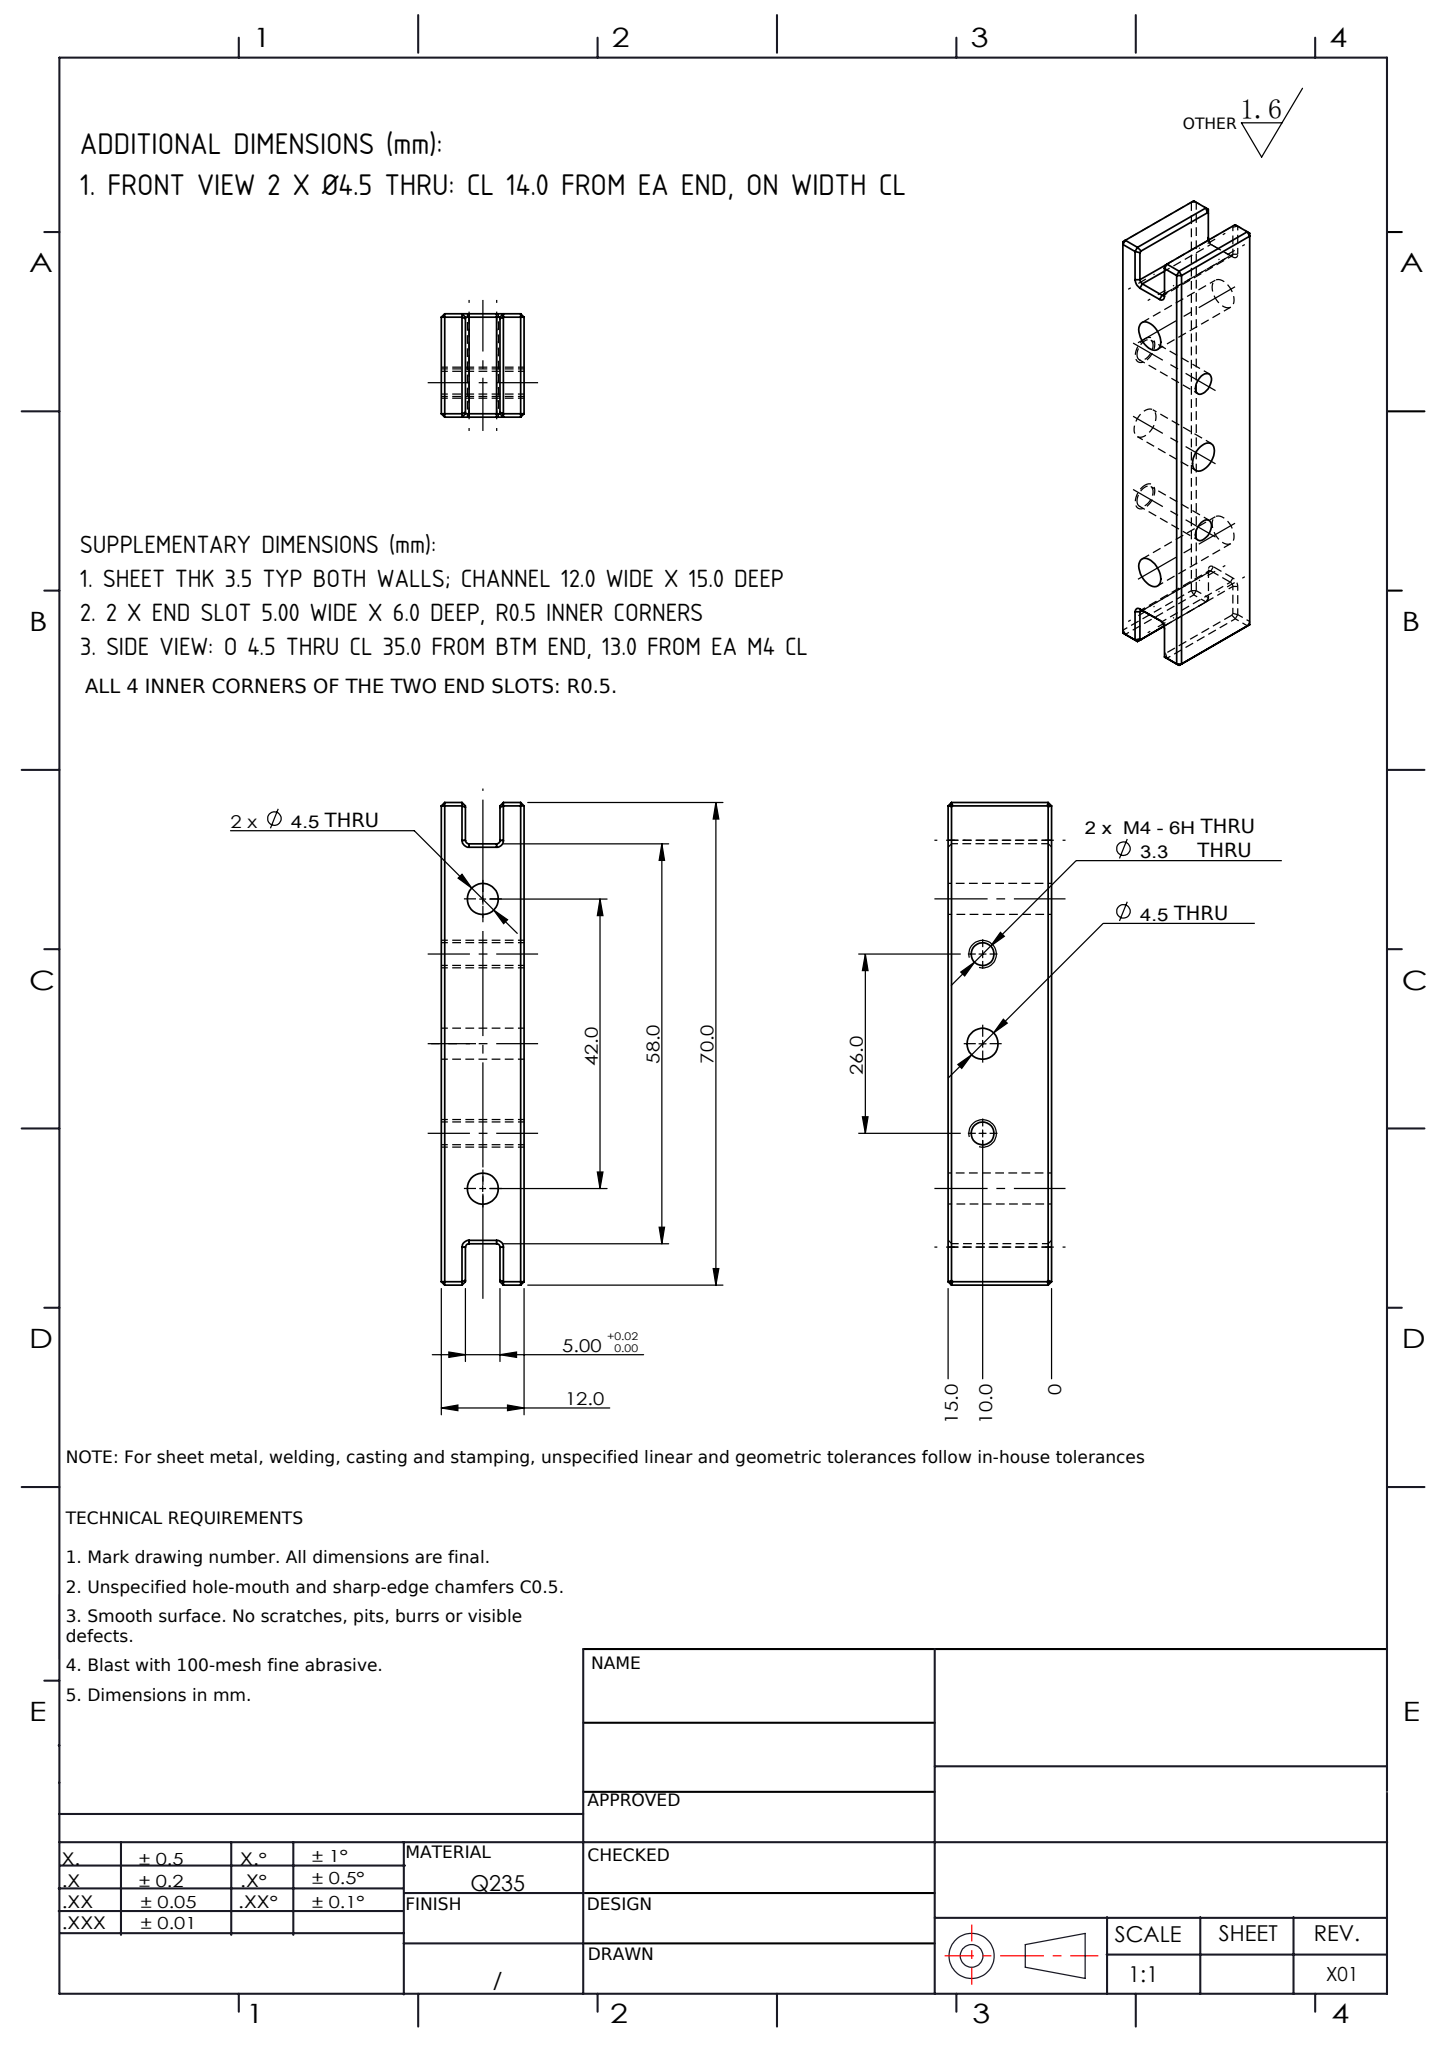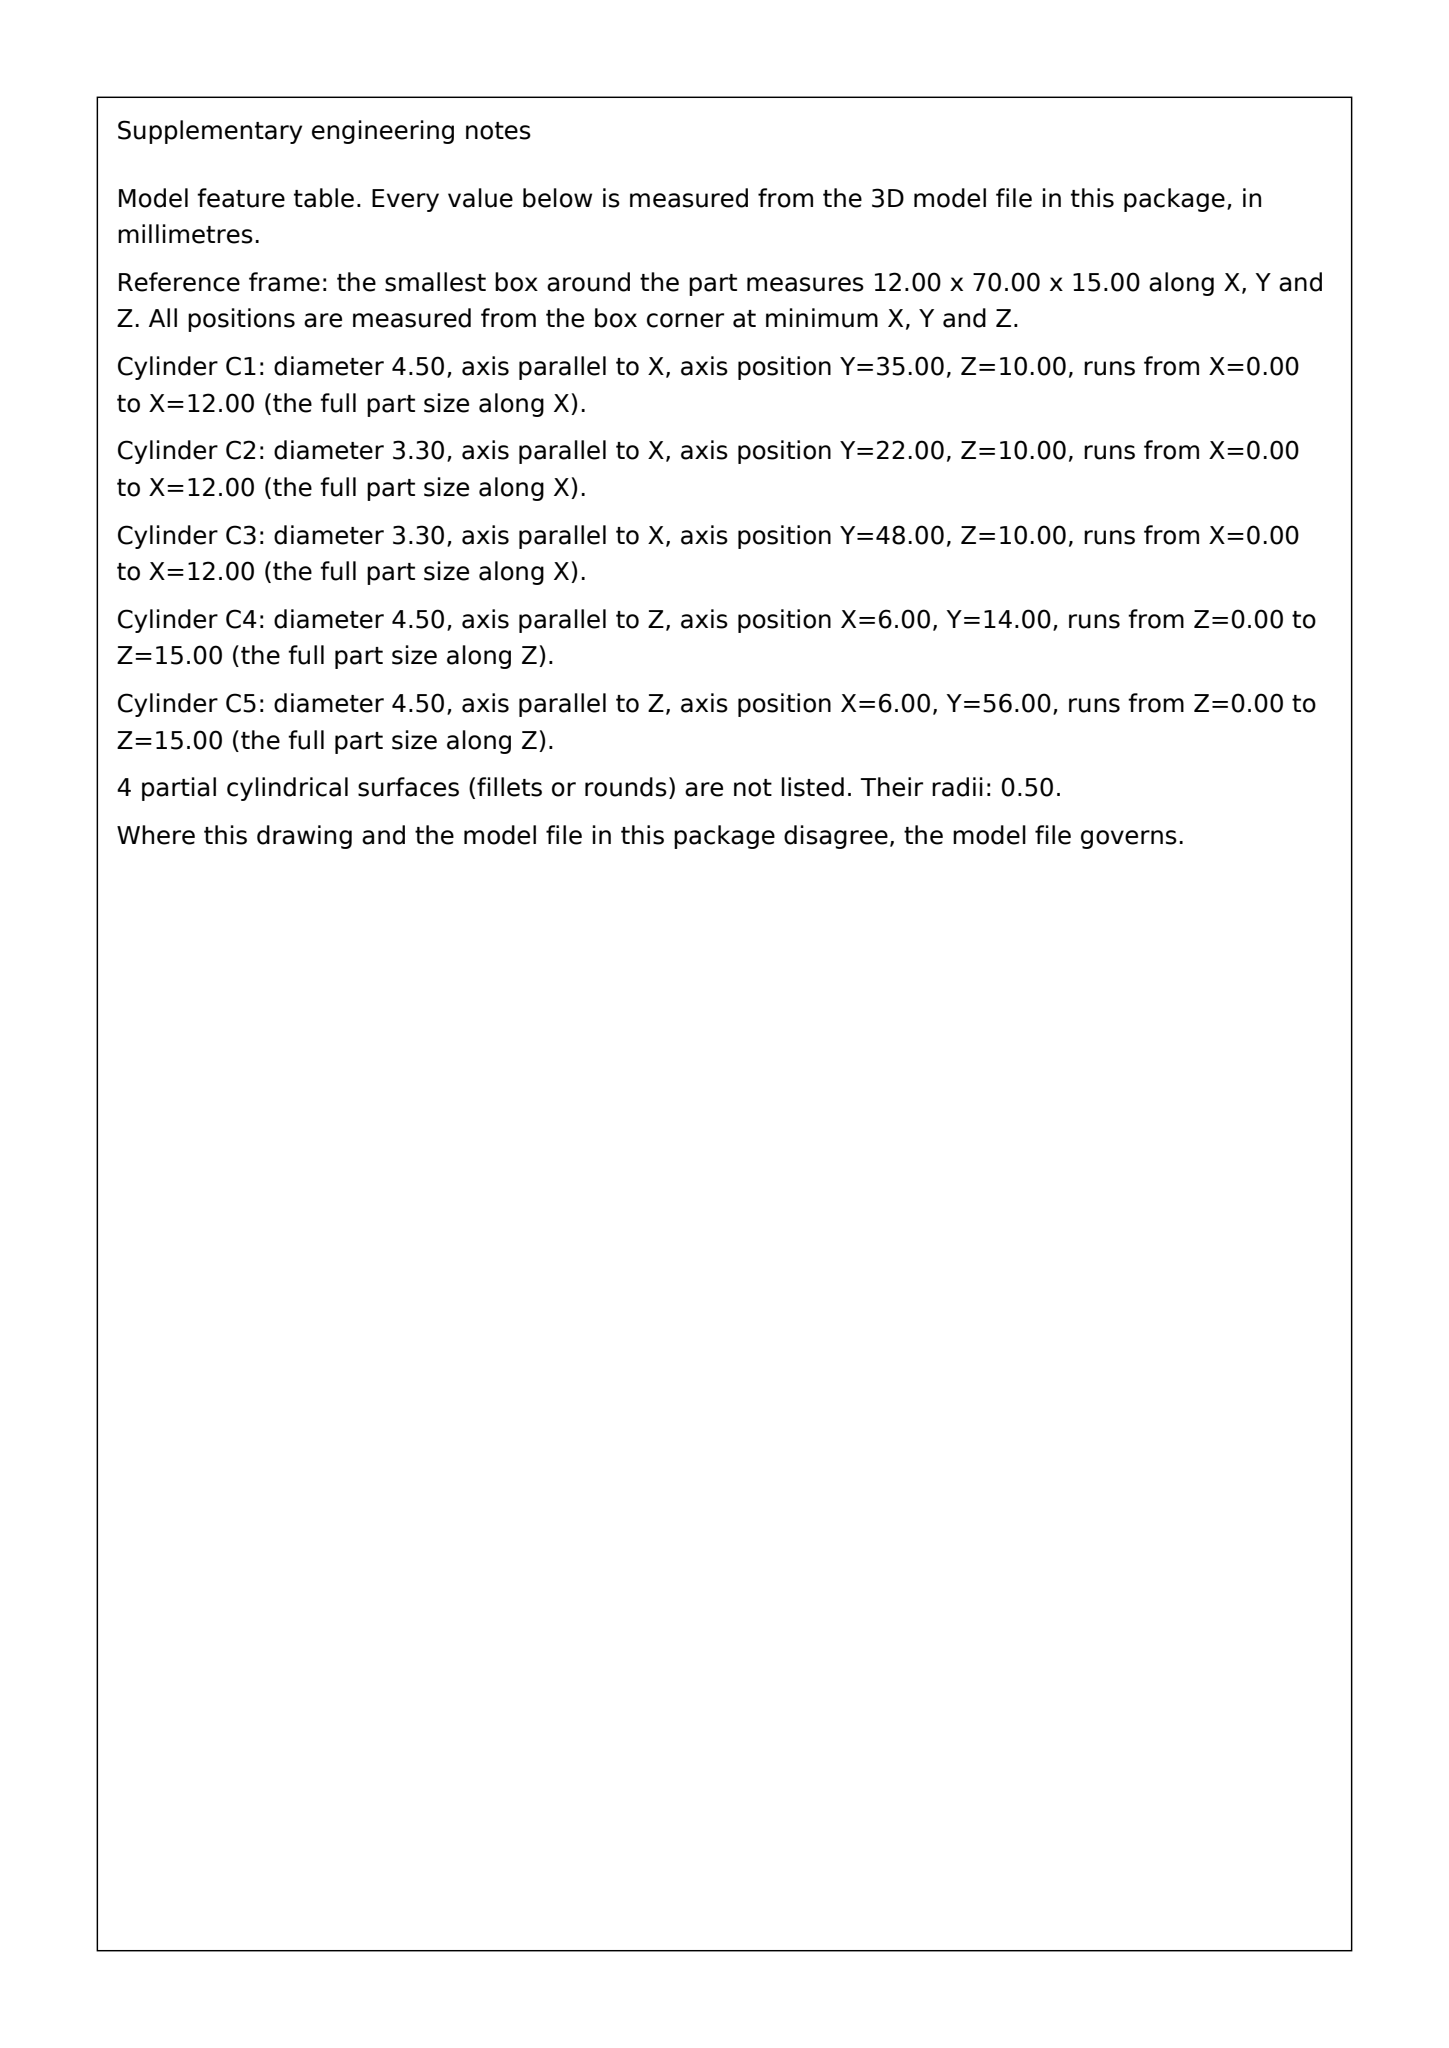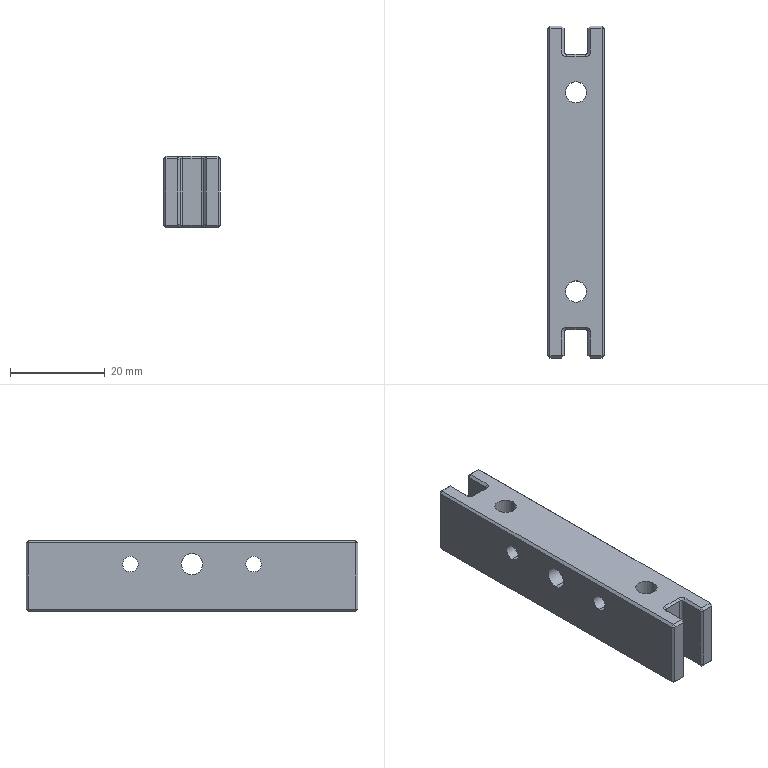Part | SolidWorks | mm | 1 solid | 84 faces | box 12 x 70 x 15 mm | volume 10769 mm3 | plane 62 | cylinder 14 | cone 8 | commonest cylinder face diameters 4.5 x6 3.3 x4 1 x4
build123d program:
from build123d import *

# Parameters (mm, degrees)
SKETCH1_W            = 12
SKETCH1_H            = 70
BOSS_EXTRUDE1_DEPTH  = 15
M4_CLEARANCE_HOLE2_D = 4.5
CHAMFER1_SIZE        = 0.5
M4_CLEARANCE_HOLE1_D = 4.5
SKETCH6_W            = 5
SKETCH6_H            = 12
CUT_EXTRUDE1_DEPTH   = 39.549
M4_TAPPED_HOLE2_D    = 3.3
FILLET1_R            = 0.5
CHAMFER2_SIZE        = 0.5


with BuildPart() as part:
    # Sketch1 → Boss-Extrude1 (new body)
    with BuildSketch(Plane.XY):
        Rectangle(SKETCH1_W, SKETCH1_H)
    extrude(amount=BOSS_EXTRUDE1_DEPTH)

    # M4 Clearance Hole2 (through all)
    with Locations(Plane.XY.offset(15)):
        with Locations((0, 21), (0, -21)):
            Hole(M4_CLEARANCE_HOLE2_D / 2)

    # Chamfer1
    chamfer1_edges = [part.edges().sort_by_distance(p)[0] for p in [
        (6, 0, 15),
        (0, 35, 15),
        (-6, 0, 15),
        (0, 35, 0),
        (6, 0, 0),
        (0, -35, 0),
        (-6, 0, 0),
        (0, -35, 15),
        (-6, 35, 7.5),
        (6, 35, 7.5),
        (6, -35, 7.5),
        (-6, -35, 7.5),
    ]]
    chamfer(chamfer1_edges, length=CHAMFER1_SIZE)

    # M4 Clearance Hole1 (through all)
    with Locations(Plane.ZY.offset(6)):
        with Locations((10, 0)):
            Hole(M4_CLEARANCE_HOLE1_D / 2)

    # Sketch6 → Cut-Extrude1 (cut, through all)
    with BuildSketch(Plane.XY.offset(15)):
        with Locations((0, 35)):
            Rectangle(SKETCH6_W, SKETCH6_H)
        with Locations((0, -35)):
            Rectangle(SKETCH6_W, SKETCH6_H)
    extrude(amount=-CUT_EXTRUDE1_DEPTH, mode=Mode.SUBTRACT)

    # M4 Tapped Hole2 (through all)
    with Locations(Plane.ZY.offset(6)):
        with Locations((10, 13), (10, -13)):
            Hole(M4_TAPPED_HOLE2_D / 2)

    # Fillet1
    fillet1_edges = [part.edges().sort_by_distance(p)[0] for p in [
        (-2.5, -29, 7.5),
        (2.5, -29, 7.5),
        (-2.5, 29, 7.5),
        (2.5, 29, 7.5),
    ]]
    fillet(fillet1_edges, radius=FILLET1_R)

    # Chamfer2
    chamfer2_edges = [part.edges().sort_by_distance(p)[0] for p in [
        (-2.5, -35, 7.5),
        (2.5, -32, 0),
        (2.5, -35, 7.5),
        (2.5, -32, 15),
        (-2.5, -32, 0),
        (-2.5, -32, 15),
        (0, -29, 15),
        (0, -29, 0),
        (0, 29, 15),
        (0, 29, 0),
        (2.5, 32, 0),
        (2.5, 32, 15),
        (-2.354, -29.146, 15),
        (-2.354, -29.146, 0),
        (2.354, -29.146, 15),
        (2.354, -29.146, 0),
        (-2.354, 29.146, 15),
        (-2.354, 29.146, 0),
        (2.354, 29.146, 15),
        (2.354, 29.146, 0),
        (2.5, 34.75, 14.75),
        (-2.5, 34.75, 14.75),
        (-2.5, 34.75, 0.25),
        (2.5, 34.75, 0.25),
        (-2.5, 32, 0),
        (-2.5, 35, 7.5),
        (2.5, 35, 7.5),
        (-2.5, 32, 15),
        (2.5, -34.75, 14.75),
        (-2.5, -34.75, 14.75),
        (-2.5, -34.75, 0.25),
        (2.5, -34.75, 0.25),
    ]]
    chamfer(chamfer2_edges, length=CHAMFER2_SIZE)


solid = part.part